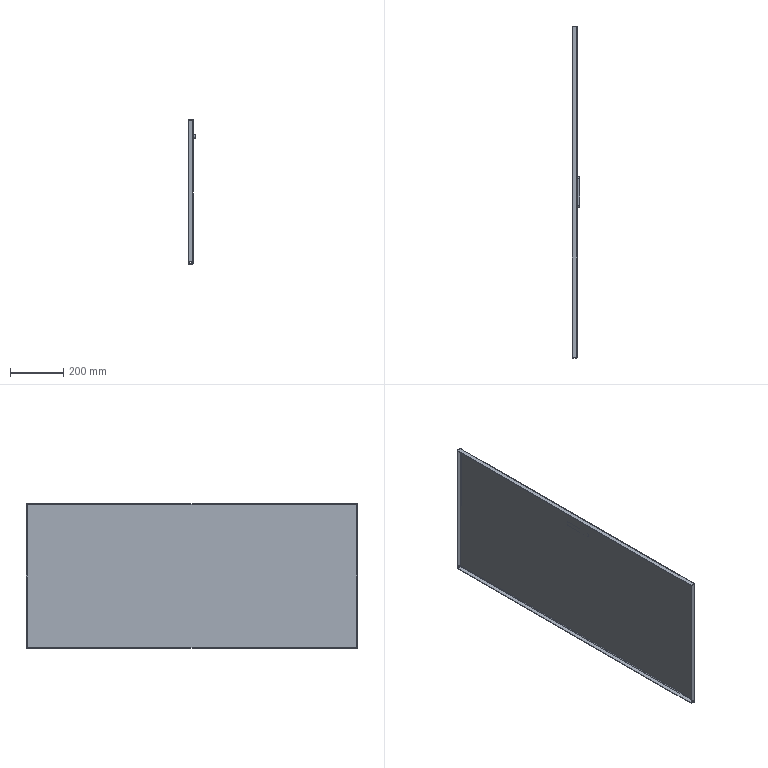Component | SolidWorks | FrontDoor-1 | 1 solid | 51 faces | volume 1494746 mm3 | plane 25 | cylinder 16 | spline 8 | torus 2 | commonest cylinder face diameters 8 x8 4 x6 16 x2